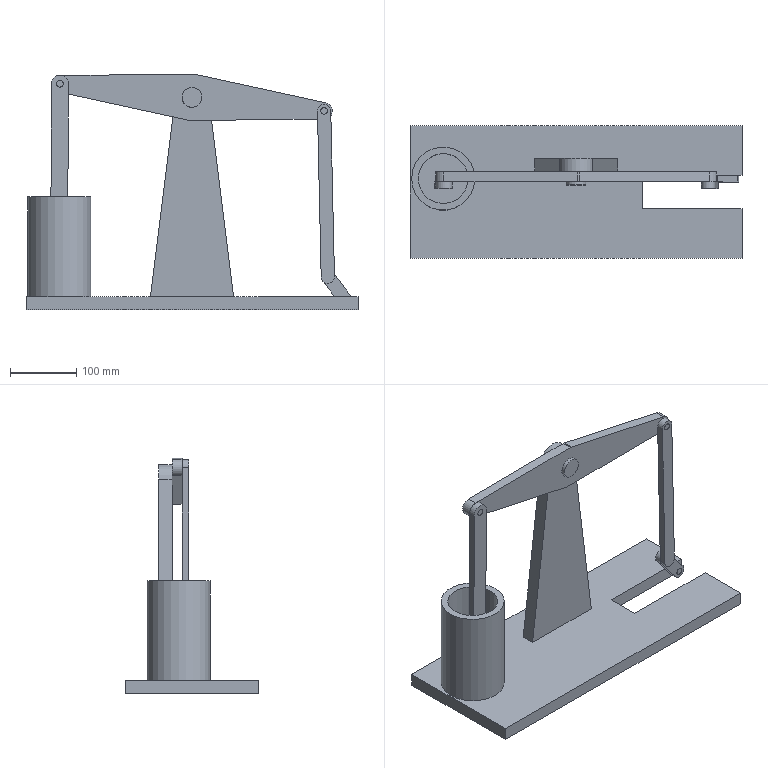Assembly | NX | mm | 7 component files | 7 solids | 73 faces | box 500 x 200 x 354.81 mm | volume 3279584 mm3 | plane 46 | cylinder 27 | commonest cylinder face diameters 10 x10 20 x7 25 x2 30 x2 25.491 x2 75 x2 50 x1 95 x1
Bill of materials:
unnamed part 1 | 1 |  | Plain hollow cylinder (tube/sleeve) with a concentric through-bore and flat ends.
unnamed part 2 | 1 |  | Flat link plate with fully rounded (obround) ends and a round through-hole near each end.
unnamed part 3 | 1 |  | Rectangular flat base plate with an open-ended rectangular slot cut in from one end, carrying a tapered upright fin with a rounded top; a short cylindrical pin/boss projects sideways from the top of the fin, and a small pin-like feature is visible near the slot end.
unnamed part 4 | 1 |  | Flat lever/arm plate in a long diamond shape, widest at the middle, with a central round through-hole and rounded narrow ends; each end has a short cylindrical pin sticking out on the same face.
unnamed part 5 | 1 |  | Long, thin, flat bar with rounded ends, a small round through-hole near one end, and a short cylindrical pin sticking out from one face near the other end.
unnamed part 6 | 1 |  | Long, thin, flat bar with rounded ends, a small round through-hole near one end, and a short cylindrical pin sticking out from one face near the other end. Very similar to unnamed part 5, but drawn slightly tilted in plan.
unnamed part 7 | 1 |  | Circular flat disc base with a single upright rectangular tab at its center; the tab has a rounded top and a round through-hole (an eye/lug).
Mates:
1. touch align | 02 1 face | stand 1 face
2. touch align | 02 1 face | stand 1 face
3. touch align | 04 1 face | stand 1 face
4. touch align | 04 1 face | stand 1 face
5. fix | stand 1 component
6. fix | stand 1 component
7. touch align | 03 1 face | 04 1 face
8. touch align | 03 1 face | 04 1 face
9. touch align | 03 1 | 02 1 face
10. touch align | 07 1 face | 02 1 face
11. touch align | 07 1 face | 02 1 face
12. touch align | circle 1 face | stand 1 face
13. distance | circle 1 face | stand 1 face
14. touch align | circle_piston 1 face | circle 1 face
15. touch align | circle_piston 1 face | 07 1 face
16. touch align | circle_piston 1 face | 07 1 face